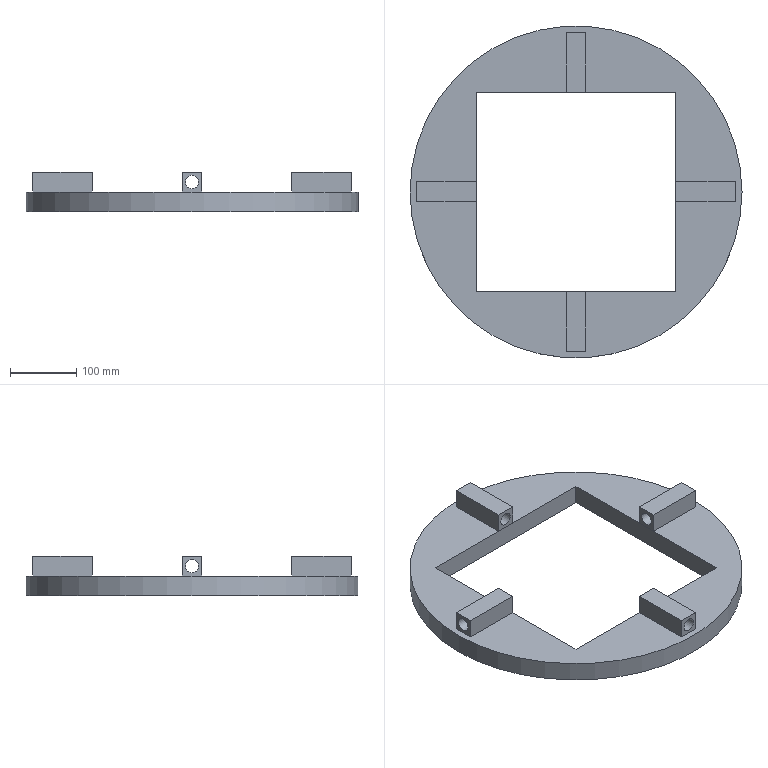Component | NX | MODEL1 | 5 solids | 35 faces | volume 3401389 mm3 | plane 30 | cylinder 5 | commonest cylinder face diameters 20 x4 500 x1